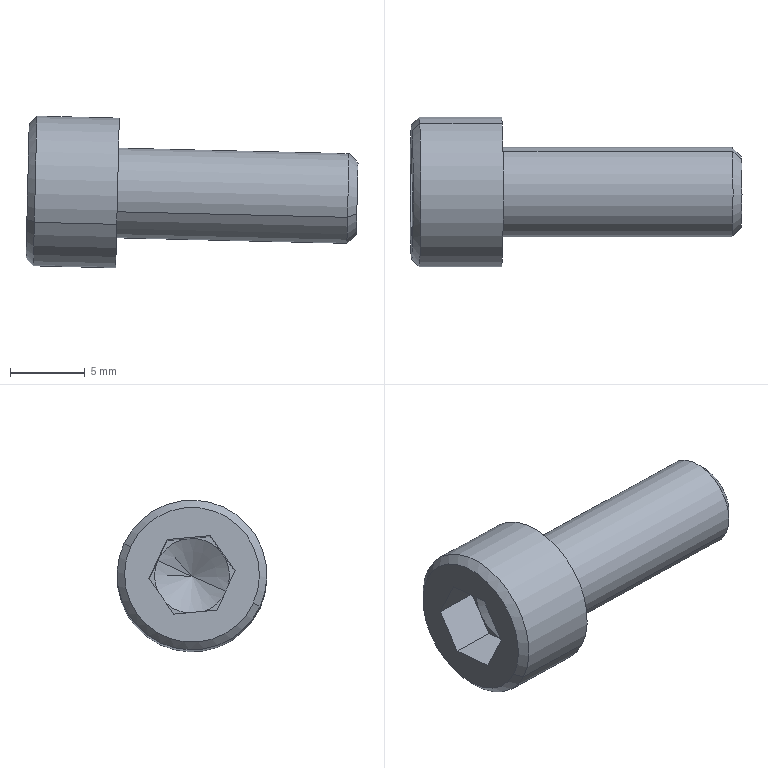Component | SolidWorks | 2012MB0201-1_ASideDoor-1-1_HexSocketHeadCapScrewM6-16FerricOxide-1 | 1 solid | 25 faces | box 22.16 x 10 x 10.13 mm | volume 842 mm3 | plane 15 | cone 6 | cylinder 4 | commonest cylinder face diameters 6 x2 10 x2 | material SCM435
STEP:
#1=CARTESIAN_POINT('',(-48.734,38.787,-7.122));
#2=VERTEX_POINT('',#1);
#3=CARTESIAN_POINT('',(-48.732,38.957,-7.043));
#4=VERTEX_POINT('',#3);
#5=CARTESIAN_POINT('',(-48.733,38.872,-7.083));
#6=DIRECTION('',(0.9997,0.,-0.02392));
#7=DIRECTION('',(0.02173,-0.4184,0.908));
#8=AXIS2_PLACEMENT_3D('',#5,#6,#7);
#9=CIRCLE('',#8,0.0939);
#10=EDGE_CURVE('',#2,#4,#9,.T.);
#11=ORIENTED_EDGE('',*,*,#10,.F.);
#12=CARTESIAN_POINT('',(-48.758,38.765,-7.131));
#13=VERTEX_POINT('',#12);
#14=CARTESIAN_POINT('',(-48.734,38.787,-7.122));
#15=DIRECTION('',(-0.714,-0.6422,-0.2789));
#16=VECTOR('',#15,39.37);
#17=LINE('',#14,#16);
#18=EDGE_CURVE('',#2,#13,#17,.T.);
#19=ORIENTED_EDGE('',*,*,#18,.T.);
#20=CARTESIAN_POINT('',(-48.756,38.979,-7.033));
#21=VERTEX_POINT('',#20);
#22=CARTESIAN_POINT('',(-48.757,38.872,-7.082));
#23=DIRECTION('',(-0.9997,-0.,0.02392));
#24=DIRECTION('',(0.01001,0.9083,0.4183));
#25=AXIS2_PLACEMENT_3D('',#22,#23,#24);
#26=CIRCLE('',#25,0.1181);
#27=EDGE_CURVE('',#21,#13,#26,.T.);
#28=ORIENTED_EDGE('',*,*,#27,.F.);
#29=CARTESIAN_POINT('',(-48.732,38.957,-7.043));
#30=DIRECTION('',(-0.6998,0.6422,0.3127));
#31=VECTOR('',#30,39.37);
#32=LINE('',#29,#31);
#33=EDGE_CURVE('',#4,#21,#32,.T.);
#34=ORIENTED_EDGE('',*,*,#33,.F.);
#35=EDGE_LOOP('',(#11,#19,#28,#34));
#36=FACE_OUTER_BOUND('',#35,.T.);
#37=CARTESIAN_POINT('',(-48.733,38.872,-7.083));
#38=DIRECTION('',(-0.9997,-0.,0.02392));
#39=DIRECTION('',(0.01001,0.9083,0.4183));
#40=AXIS2_PLACEMENT_3D('',#37,#38,#39);
#41=CONICAL_SURFACE('',#40,0.0939,0.7854);
#42=ADVANCED_FACE('',(#36),#41,.T.);
#43=ORIENTED_EDGE('',*,*,#27,.T.);
#44=CARTESIAN_POINT('',(-49.364,38.765,-7.117));
#45=VERTEX_POINT('',#44);
#46=CARTESIAN_POINT('',(-45.428,38.765,-7.211));
#47=DIRECTION('',(-0.9997,-0.,0.02392));
#48=VECTOR('',#47,39.37);
#49=LINE('',#46,#48);
#50=EDGE_CURVE('',#13,#45,#49,.T.);
#51=ORIENTED_EDGE('',*,*,#50,.T.);
#52=CARTESIAN_POINT('',(-49.361,38.979,-7.018));
#53=VERTEX_POINT('',#52);
#54=CARTESIAN_POINT('',(-49.362,38.872,-7.068));
#55=DIRECTION('',(0.9997,0.,-0.02392));
#56=DIRECTION('',(0.01001,0.9083,0.4183));
#57=AXIS2_PLACEMENT_3D('',#54,#55,#56);
#58=CIRCLE('',#57,0.1181);
#59=EDGE_CURVE('',#45,#53,#58,.T.);
#60=ORIENTED_EDGE('',*,*,#59,.T.);
#61=CARTESIAN_POINT('',(-45.425,38.979,-7.112));
#62=DIRECTION('',(-0.9997,-0.,0.02392));
#63=VECTOR('',#62,39.37);
#64=LINE('',#61,#63);
#65=EDGE_CURVE('',#21,#53,#64,.T.);
#66=ORIENTED_EDGE('',*,*,#65,.F.);
#67=EDGE_LOOP('',(#43,#51,#60,#66));
#68=FACE_OUTER_BOUND('',#67,.T.);
#69=CARTESIAN_POINT('',(-45.427,38.872,-7.162));
#70=DIRECTION('',(-0.9997,-0.,0.02392));
#71=DIRECTION('',(0.01001,0.9083,0.4183));
#72=AXIS2_PLACEMENT_3D('',#69,#70,#71);
#73=CYLINDRICAL_SURFACE('',#72,0.1181);
#74=ADVANCED_FACE('',(#68),#73,.T.);
#75=CARTESIAN_POINT('',(-49.36,39.051,-6.985));
#76=VERTEX_POINT('',#75);
#77=CARTESIAN_POINT('',(-49.364,38.693,-7.15));
#78=VERTEX_POINT('',#77);
#79=CARTESIAN_POINT('',(-49.362,38.872,-7.068));
#80=DIRECTION('',(-0.9997,-0.,0.02392));
#81=DIRECTION('',(0.01001,0.9083,0.4183));
#82=AXIS2_PLACEMENT_3D('',#79,#80,#81);
#83=CIRCLE('',#82,0.1969);
#84=EDGE_CURVE('',#76,#78,#83,.T.);
#85=ORIENTED_EDGE('',*,*,#84,.T.);
#86=CARTESIAN_POINT('',(-49.581,38.693,-7.145));
#87=VERTEX_POINT('',#86);
#88=CARTESIAN_POINT('',(-49.364,38.693,-7.15));
#89=DIRECTION('',(-0.9997,-0.,0.02392));
#90=VECTOR('',#89,39.37);
#91=LINE('',#88,#90);
#92=EDGE_CURVE('',#78,#87,#91,.T.);
#93=ORIENTED_EDGE('',*,*,#92,.T.);
#94=CARTESIAN_POINT('',(-49.577,39.051,-6.98));
#95=VERTEX_POINT('',#94);
#96=CARTESIAN_POINT('',(-49.579,38.872,-7.062));
#97=DIRECTION('',(0.9997,0.,-0.02392));
#98=DIRECTION('',(0.01001,0.9083,0.4183));
#99=AXIS2_PLACEMENT_3D('',#96,#97,#98);
#100=CIRCLE('',#99,0.1969);
#101=EDGE_CURVE('',#87,#95,#100,.T.);
#102=ORIENTED_EDGE('',*,*,#101,.T.);
#103=CARTESIAN_POINT('',(-49.36,39.051,-6.985));
#104=DIRECTION('',(-0.9997,-0.,0.02392));
#105=VECTOR('',#104,39.37);
#106=LINE('',#103,#105);
#107=EDGE_CURVE('',#76,#95,#106,.T.);
#108=ORIENTED_EDGE('',*,*,#107,.F.);
#109=EDGE_LOOP('',(#85,#93,#102,#108));
#110=FACE_OUTER_BOUND('',#109,.T.);
#111=CARTESIAN_POINT('',(-49.362,38.872,-7.068));
#112=DIRECTION('',(-0.9997,-0.,0.02392));
#113=DIRECTION('',(0.01001,0.9083,0.4183));
#114=AXIS2_PLACEMENT_3D('',#111,#112,#113);
#115=CYLINDRICAL_SURFACE('',#114,0.1969);
#116=ADVANCED_FACE('',(#110),#115,.T.);
#117=CARTESIAN_POINT('',(-49.6,38.711,-7.136));
#118=VERTEX_POINT('',#117);
#119=CARTESIAN_POINT('',(-49.597,39.033,-6.988));
#120=VERTEX_POINT('',#119);
#121=CARTESIAN_POINT('',(-49.599,38.872,-7.062));
#122=DIRECTION('',(0.9997,0.,-0.02392));
#123=DIRECTION('',(-0.01001,-0.9083,-0.4183));
#124=AXIS2_PLACEMENT_3D('',#121,#122,#123);
#125=CIRCLE('',#124,0.1772);
#126=EDGE_CURVE('',#118,#120,#125,.T.);
#127=ORIENTED_EDGE('',*,*,#126,.T.);
#128=CARTESIAN_POINT('',(-49.577,39.051,-6.98));
#129=DIRECTION('',(0.714,0.6422,0.2789));
#130=VECTOR('',#129,39.37);
#131=LINE('',#128,#130);
#132=EDGE_CURVE('',#120,#95,#131,.T.);
#133=ORIENTED_EDGE('',*,*,#132,.T.);
#134=ORIENTED_EDGE('',*,*,#101,.F.);
#135=CARTESIAN_POINT('',(-49.581,38.693,-7.145));
#136=DIRECTION('',(0.6998,-0.6422,-0.3127));
#137=VECTOR('',#136,39.37);
#138=LINE('',#135,#137);
#139=EDGE_CURVE('',#118,#87,#138,.T.);
#140=ORIENTED_EDGE('',*,*,#139,.F.);
#141=EDGE_LOOP('',(#127,#133,#134,#140));
#142=FACE_OUTER_BOUND('',#141,.T.);
#143=CARTESIAN_POINT('',(-49.579,38.872,-7.062));
#144=DIRECTION('',(0.9997,0.,-0.02392));
#145=DIRECTION('',(-0.01001,-0.9083,-0.4183));
#146=AXIS2_PLACEMENT_3D('',#143,#144,#145);
#147=CONICAL_SURFACE('',#146,0.1969,0.7854);
#148=ADVANCED_FACE('',(#142),#147,.T.);
#149=CARTESIAN_POINT('',(-49.424,38.872,-7.066));
#150=VERTEX_POINT('',#149);
#151=CARTESIAN_POINT('',(-49.48,38.961,-7.024));
#152=VERTEX_POINT('',#151);
#153=CARTESIAN_POINT('',(-49.48,38.961,-7.024));
#154=DIRECTION('',(-0.4912,0.7866,0.3742));
#155=VECTOR('',#154,39.37);
#156=LINE('',#153,#155);
#157=EDGE_CURVE('',#150,#152,#156,.T.);
#158=ORIENTED_EDGE('',*,*,#157,.F.);
#159=CARTESIAN_POINT('',(-49.482,38.783,-7.106));
#160=VERTEX_POINT('',#159);
#161=CARTESIAN_POINT('',(-49.482,38.783,-7.106));
#162=DIRECTION('',(-0.5085,-0.7866,-0.3503));
#163=VECTOR('',#162,39.37);
#164=LINE('',#161,#163);
#165=EDGE_CURVE('',#150,#160,#164,.T.);
#166=ORIENTED_EDGE('',*,*,#165,.T.);
#167=CARTESIAN_POINT('',(-49.479,38.792,-7.008));
#168=VERTEX_POINT('',#167);
#169=CARTESIAN_POINT('',(-49.481,38.872,-7.065));
#170=DIRECTION('',(0.9997,0.,-0.02392));
#171=DIRECTION('',(0.01001,0.9083,0.4183));
#172=AXIS2_PLACEMENT_3D('',#169,#170,#171);
#173=CIRCLE('',#172,0.09843);
#174=EDGE_CURVE('',#168,#160,#173,.T.);
#175=ORIENTED_EDGE('',*,*,#174,.F.);
#176=CARTESIAN_POINT('',(-49.478,38.881,-6.967));
#177=VERTEX_POINT('',#176);
#178=CARTESIAN_POINT('',(-49.481,38.872,-7.065));
#179=DIRECTION('',(0.9997,0.,-0.02392));
#180=DIRECTION('',(0.01001,0.9083,0.4183));
#181=AXIS2_PLACEMENT_3D('',#178,#179,#180);
#182=CIRCLE('',#181,0.09843);
#183=EDGE_CURVE('',#177,#168,#182,.T.);
#184=ORIENTED_EDGE('',*,*,#183,.F.);
#185=CARTESIAN_POINT('',(-49.481,38.872,-7.065));
#186=DIRECTION('',(0.9997,0.,-0.02392));
#187=DIRECTION('',(0.01001,0.9083,0.4183));
#188=AXIS2_PLACEMENT_3D('',#185,#186,#187);
#189=CIRCLE('',#188,0.09843);
#190=EDGE_CURVE('',#152,#177,#189,.T.);
#191=ORIENTED_EDGE('',*,*,#190,.F.);
#192=EDGE_LOOP('',(#158,#166,#175,#184,#191));
#193=FACE_OUTER_BOUND('',#192,.T.);
#194=CARTESIAN_POINT('',(-49.481,38.872,-7.065));
#195=DIRECTION('',(-0.9997,-0.,0.02392));
#196=DIRECTION('',(0.01001,0.9083,0.4183));
#197=AXIS2_PLACEMENT_3D('',#194,#195,#196);
#198=CONICAL_SURFACE('',#197,0.09843,1.047);
#199=ADVANCED_FACE('',(#193),#198,.F.);
#200=ORIENTED_EDGE('',*,*,#50,.F.);
#201=CARTESIAN_POINT('',(-48.757,38.872,-7.082));
#202=DIRECTION('',(-0.9997,-0.,0.02392));
#203=DIRECTION('',(0.01001,0.9083,0.4183));
#204=AXIS2_PLACEMENT_3D('',#201,#202,#203);
#205=CIRCLE('',#204,0.1181);
#206=EDGE_CURVE('',#13,#21,#205,.T.);
#207=ORIENTED_EDGE('',*,*,#206,.T.);
#208=ORIENTED_EDGE('',*,*,#65,.T.);
#209=CARTESIAN_POINT('',(-49.362,38.872,-7.068));
#210=DIRECTION('',(0.9997,0.,-0.02392));
#211=DIRECTION('',(0.01001,0.9083,0.4183));
#212=AXIS2_PLACEMENT_3D('',#209,#210,#211);
#213=CIRCLE('',#212,0.1181);
#214=EDGE_CURVE('',#53,#45,#213,.T.);
#215=ORIENTED_EDGE('',*,*,#214,.T.);
#216=EDGE_LOOP('',(#200,#207,#208,#215));
#217=FACE_OUTER_BOUND('',#216,.T.);
#218=CARTESIAN_POINT('',(-45.427,38.872,-7.162));
#219=DIRECTION('',(-0.9997,-0.,0.02392));
#220=DIRECTION('',(0.01001,0.9083,0.4183));
#221=AXIS2_PLACEMENT_3D('',#218,#219,#220);
#222=CYLINDRICAL_SURFACE('',#221,0.1181);
#223=ADVANCED_FACE('',(#217),#222,.T.);
#224=ORIENTED_EDGE('',*,*,#84,.F.);
#225=CARTESIAN_POINT('',(-49.362,38.872,-7.068));
#226=DIRECTION('',(-0.9997,-0.,0.02392));
#227=DIRECTION('',(0.01001,0.9083,0.4183));
#228=AXIS2_PLACEMENT_3D('',#225,#226,#227);
#229=CIRCLE('',#228,0.1969);
#230=EDGE_CURVE('',#78,#76,#229,.T.);
#231=ORIENTED_EDGE('',*,*,#230,.F.);
#232=EDGE_LOOP('',(#224,#231));
#233=FACE_OUTER_BOUND('',#232,.T.);
#234=ORIENTED_EDGE('',*,*,#214,.F.);
#235=ORIENTED_EDGE('',*,*,#59,.F.);
#236=EDGE_LOOP('',(#234,#235));
#237=FACE_BOUND('',#236,.T.);
#238=CARTESIAN_POINT('',(-49.367,38.954,-7.246));
#239=DIRECTION('',(-0.9997,-0.,0.02392));
#240=DIRECTION('',(0.01001,0.9083,0.4183));
#241=AXIS2_PLACEMENT_3D('',#238,#239,#240);
#242=PLANE('',#241);
#243=ADVANCED_FACE('',(#233,#237),#242,.F.);
#244=ORIENTED_EDGE('',*,*,#92,.F.);
#245=ORIENTED_EDGE('',*,*,#230,.T.);
#246=ORIENTED_EDGE('',*,*,#107,.T.);
#247=CARTESIAN_POINT('',(-49.579,38.872,-7.062));
#248=DIRECTION('',(0.9997,0.,-0.02392));
#249=DIRECTION('',(0.01001,0.9083,0.4183));
#250=AXIS2_PLACEMENT_3D('',#247,#248,#249);
#251=CIRCLE('',#250,0.1969);
#252=EDGE_CURVE('',#95,#87,#251,.T.);
#253=ORIENTED_EDGE('',*,*,#252,.T.);
#254=EDGE_LOOP('',(#244,#245,#246,#253));
#255=FACE_OUTER_BOUND('',#254,.T.);
#256=CARTESIAN_POINT('',(-49.362,38.872,-7.068));
#257=DIRECTION('',(-0.9997,-0.,0.02392));
#258=DIRECTION('',(0.01001,0.9083,0.4183));
#259=AXIS2_PLACEMENT_3D('',#256,#257,#258);
#260=CYLINDRICAL_SURFACE('',#259,0.1969);
#261=ADVANCED_FACE('',(#255),#260,.T.);
#262=ORIENTED_EDGE('',*,*,#132,.F.);
#263=CARTESIAN_POINT('',(-49.599,38.872,-7.062));
#264=DIRECTION('',(0.9997,0.,-0.02392));
#265=DIRECTION('',(-0.01001,-0.9083,-0.4183));
#266=AXIS2_PLACEMENT_3D('',#263,#264,#265);
#267=CIRCLE('',#266,0.1772);
#268=EDGE_CURVE('',#120,#118,#267,.T.);
#269=ORIENTED_EDGE('',*,*,#268,.T.);
#270=ORIENTED_EDGE('',*,*,#139,.T.);
#271=ORIENTED_EDGE('',*,*,#252,.F.);
#272=EDGE_LOOP('',(#262,#269,#270,#271));
#273=FACE_OUTER_BOUND('',#272,.T.);
#274=CARTESIAN_POINT('',(-49.579,38.872,-7.062));
#275=DIRECTION('',(0.9997,0.,-0.02392));
#276=DIRECTION('',(-0.01001,-0.9083,-0.4183));
#277=AXIS2_PLACEMENT_3D('',#274,#275,#276);
#278=CONICAL_SURFACE('',#277,0.1969,0.7854);
#279=ADVANCED_FACE('',(#273),#278,.T.);
#280=CARTESIAN_POINT('',(-49.598,38.759,-7.051));
#281=VERTEX_POINT('',#280);
#282=CARTESIAN_POINT('',(-49.596,38.825,-6.959));
#283=VERTEX_POINT('',#282);
#284=CARTESIAN_POINT('',(-49.598,38.759,-7.051));
#285=DIRECTION('',(0.01953,0.5774,0.8163));
#286=VECTOR('',#285,39.37);
#287=LINE('',#284,#286);
#288=EDGE_CURVE('',#281,#283,#287,.T.);
#289=ORIENTED_EDGE('',*,*,#288,.F.);
#290=CARTESIAN_POINT('',(-49.601,38.806,-7.155));
#291=VERTEX_POINT('',#290);
#292=CARTESIAN_POINT('',(-49.6,38.783,-7.103));
#293=DIRECTION('',(0.02173,-0.4184,0.908));
#294=VECTOR('',#293,39.37);
#295=LINE('',#292,#294);
#296=EDGE_CURVE('',#291,#281,#295,.T.);
#297=ORIENTED_EDGE('',*,*,#296,.F.);
#298=CARTESIAN_POINT('',(-49.601,38.92,-7.165));
#299=VERTEX_POINT('',#298);
#300=CARTESIAN_POINT('',(-49.601,38.92,-7.165));
#301=DIRECTION('',(0.002195,-0.9958,0.09174));
#302=VECTOR('',#301,39.37);
#303=LINE('',#300,#302);
#304=EDGE_CURVE('',#299,#291,#303,.T.);
#305=ORIENTED_EDGE('',*,*,#304,.F.);
#306=CARTESIAN_POINT('',(-49.599,38.985,-7.072));
#307=VERTEX_POINT('',#306);
#308=CARTESIAN_POINT('',(-49.599,38.985,-7.072));
#309=DIRECTION('',(-0.01953,-0.5774,-0.8163));
#310=VECTOR('',#309,39.37);
#311=LINE('',#308,#310);
#312=EDGE_CURVE('',#307,#299,#311,.T.);
#313=ORIENTED_EDGE('',*,*,#312,.F.);
#314=CARTESIAN_POINT('',(-49.596,38.938,-6.969));
#315=VERTEX_POINT('',#314);
#316=CARTESIAN_POINT('',(-49.598,38.961,-7.021));
#317=DIRECTION('',(-0.02173,0.4184,-0.908));
#318=VECTOR('',#317,39.37);
#319=LINE('',#316,#318);
#320=EDGE_CURVE('',#315,#307,#319,.T.);
#321=ORIENTED_EDGE('',*,*,#320,.F.);
#322=CARTESIAN_POINT('',(-49.596,38.825,-6.959));
#323=DIRECTION('',(-0.002195,0.9958,-0.09174));
#324=VECTOR('',#323,39.37);
#325=LINE('',#322,#324);
#326=EDGE_CURVE('',#283,#315,#325,.T.);
#327=ORIENTED_EDGE('',*,*,#326,.F.);
#328=EDGE_LOOP('',(#289,#297,#305,#313,#321,#327));
#329=FACE_BOUND('',#328,.T.);
#330=ORIENTED_EDGE('',*,*,#126,.F.);
#331=ORIENTED_EDGE('',*,*,#268,.F.);
#332=EDGE_LOOP('',(#330,#331));
#333=FACE_OUTER_BOUND('',#332,.T.);
#334=CARTESIAN_POINT('',(-49.599,38.872,-7.062));
#335=DIRECTION('',(0.9997,0.,-0.02392));
#336=DIRECTION('',(-0.01001,-0.9083,-0.4183));
#337=AXIS2_PLACEMENT_3D('',#334,#335,#336);
#338=PLANE('',#337);
#339=ADVANCED_FACE('',(#329,#333),#338,.F.);
#340=CARTESIAN_POINT('',(-49.478,38.938,-6.972));
#341=VERTEX_POINT('',#340);
#342=CARTESIAN_POINT('',(-49.478,38.938,-6.972));
#343=DIRECTION('',(-0.9997,-0.,0.02392));
#344=VECTOR('',#343,39.37);
#345=LINE('',#342,#344);
#346=EDGE_CURVE('',#341,#315,#345,.T.);
#347=ORIENTED_EDGE('',*,*,#346,.F.);
#348=CARTESIAN_POINT('',(-49.478,38.881,-6.967));
#349=DIRECTION('',(-0.002195,0.9958,-0.09174));
#350=VECTOR('',#349,39.37);
#351=LINE('',#348,#350);
#352=EDGE_CURVE('',#177,#341,#351,.T.);
#353=ORIENTED_EDGE('',*,*,#352,.F.);
#354=CARTESIAN_POINT('',(-49.478,38.825,-6.962));
#355=VERTEX_POINT('',#354);
#356=CARTESIAN_POINT('',(-49.478,38.825,-6.962));
#357=DIRECTION('',(-0.002195,0.9958,-0.09174));
#358=VECTOR('',#357,39.37);
#359=LINE('',#356,#358);
#360=EDGE_CURVE('',#355,#177,#359,.T.);
#361=ORIENTED_EDGE('',*,*,#360,.F.);
#362=CARTESIAN_POINT('',(-49.478,38.825,-6.962));
#363=DIRECTION('',(0.9997,0.,-0.02392));
#364=VECTOR('',#363,39.37);
#365=LINE('',#362,#364);
#366=EDGE_CURVE('',#283,#355,#365,.T.);
#367=ORIENTED_EDGE('',*,*,#366,.F.);
#368=ORIENTED_EDGE('',*,*,#326,.T.);
#369=EDGE_LOOP('',(#347,#353,#361,#367,#368));
#370=FACE_OUTER_BOUND('',#369,.T.);
#371=CARTESIAN_POINT('',(-49.478,38.825,-6.962));
#372=DIRECTION('',(0.02382,0.09177,0.9955));
#373=DIRECTION('',(-0.002195,0.9958,-0.09174));
#374=AXIS2_PLACEMENT_3D('',#371,#372,#373);
#375=PLANE('',#374);
#376=ADVANCED_FACE('',(#370),#375,.F.);
#377=ORIENTED_EDGE('',*,*,#366,.T.);
#378=CARTESIAN_POINT('',(-49.479,38.792,-7.008));
#379=DIRECTION('',(0.01953,0.5774,0.8163));
#380=VECTOR('',#379,39.37);
#381=LINE('',#378,#380);
#382=EDGE_CURVE('',#168,#355,#381,.T.);
#383=ORIENTED_EDGE('',*,*,#382,.F.);
#384=CARTESIAN_POINT('',(-49.48,38.759,-7.054));
#385=VERTEX_POINT('',#384);
#386=CARTESIAN_POINT('',(-49.48,38.759,-7.054));
#387=DIRECTION('',(0.01953,0.5774,0.8163));
#388=VECTOR('',#387,39.37);
#389=LINE('',#386,#388);
#390=EDGE_CURVE('',#385,#168,#389,.T.);
#391=ORIENTED_EDGE('',*,*,#390,.F.);
#392=CARTESIAN_POINT('',(-49.48,38.759,-7.054));
#393=DIRECTION('',(0.9997,0.,-0.02392));
#394=VECTOR('',#393,39.37);
#395=LINE('',#392,#394);
#396=EDGE_CURVE('',#281,#385,#395,.T.);
#397=ORIENTED_EDGE('',*,*,#396,.F.);
#398=ORIENTED_EDGE('',*,*,#288,.T.);
#399=EDGE_LOOP('',(#377,#383,#391,#397,#398));
#400=FACE_OUTER_BOUND('',#399,.T.);
#401=CARTESIAN_POINT('',(-49.48,38.759,-7.054));
#402=DIRECTION('',(0.01381,-0.8165,0.5772));
#403=DIRECTION('',(0.01953,0.5774,0.8163));
#404=AXIS2_PLACEMENT_3D('',#401,#402,#403);
#405=PLANE('',#404);
#406=ADVANCED_FACE('',(#400),#405,.F.);
#407=ORIENTED_EDGE('',*,*,#396,.T.);
#408=CARTESIAN_POINT('',(-49.482,38.783,-7.106));
#409=DIRECTION('',(0.02173,-0.4184,0.908));
#410=VECTOR('',#409,39.37);
#411=LINE('',#408,#410);
#412=EDGE_CURVE('',#160,#385,#411,.T.);
#413=ORIENTED_EDGE('',*,*,#412,.F.);
#414=CARTESIAN_POINT('',(-49.483,38.806,-7.158));
#415=VERTEX_POINT('',#414);
#416=CARTESIAN_POINT('',(-49.482,38.783,-7.106));
#417=DIRECTION('',(0.02173,-0.4184,0.908));
#418=VECTOR('',#417,39.37);
#419=LINE('',#416,#418);
#420=EDGE_CURVE('',#415,#160,#419,.T.);
#421=ORIENTED_EDGE('',*,*,#420,.F.);
#422=CARTESIAN_POINT('',(-49.483,38.806,-7.158));
#423=DIRECTION('',(0.9997,0.,-0.02392));
#424=VECTOR('',#423,39.37);
#425=LINE('',#422,#424);
#426=EDGE_CURVE('',#291,#415,#425,.T.);
#427=ORIENTED_EDGE('',*,*,#426,.F.);
#428=ORIENTED_EDGE('',*,*,#296,.T.);
#429=EDGE_LOOP('',(#407,#413,#421,#427,#428));
#430=FACE_OUTER_BOUND('',#429,.T.);
#431=CARTESIAN_POINT('',(-49.483,38.806,-7.158));
#432=DIRECTION('',(-0.01001,-0.9083,-0.4183));
#433=DIRECTION('',(-0.9997,-0.,0.02392));
#434=AXIS2_PLACEMENT_3D('',#431,#432,#433);
#435=PLANE('',#434);
#436=ADVANCED_FACE('',(#430),#435,.F.);
#437=ORIENTED_EDGE('',*,*,#426,.T.);
#438=CARTESIAN_POINT('',(-49.483,38.863,-7.163));
#439=VERTEX_POINT('',#438);
#440=CARTESIAN_POINT('',(-49.483,38.863,-7.163));
#441=DIRECTION('',(0.002195,-0.9958,0.09174));
#442=VECTOR('',#441,39.37);
#443=LINE('',#440,#442);
#444=EDGE_CURVE('',#439,#415,#443,.T.);
#445=ORIENTED_EDGE('',*,*,#444,.F.);
#446=CARTESIAN_POINT('',(-49.483,38.92,-7.168));
#447=VERTEX_POINT('',#446);
#448=CARTESIAN_POINT('',(-49.483,38.92,-7.168));
#449=DIRECTION('',(0.002195,-0.9958,0.09174));
#450=VECTOR('',#449,39.37);
#451=LINE('',#448,#450);
#452=EDGE_CURVE('',#447,#439,#451,.T.);
#453=ORIENTED_EDGE('',*,*,#452,.F.);
#454=CARTESIAN_POINT('',(-49.483,38.92,-7.168));
#455=DIRECTION('',(0.9997,0.,-0.02392));
#456=VECTOR('',#455,39.37);
#457=LINE('',#454,#456);
#458=EDGE_CURVE('',#299,#447,#457,.T.);
#459=ORIENTED_EDGE('',*,*,#458,.F.);
#460=ORIENTED_EDGE('',*,*,#304,.T.);
#461=EDGE_LOOP('',(#437,#445,#453,#459,#460));
#462=FACE_OUTER_BOUND('',#461,.T.);
#463=CARTESIAN_POINT('',(-49.483,38.92,-7.168));
#464=DIRECTION('',(-0.02382,-0.09177,-0.9955));
#465=DIRECTION('',(0.002195,-0.9958,0.09174));
#466=AXIS2_PLACEMENT_3D('',#463,#464,#465);
#467=PLANE('',#466);
#468=ADVANCED_FACE('',(#462),#467,.F.);
#469=ORIENTED_EDGE('',*,*,#458,.T.);
#470=CARTESIAN_POINT('',(-49.482,38.952,-7.122));
#471=VERTEX_POINT('',#470);
#472=CARTESIAN_POINT('',(-49.482,38.952,-7.122));
#473=DIRECTION('',(-0.01953,-0.5774,-0.8163));
#474=VECTOR('',#473,39.37);
#475=LINE('',#472,#474);
#476=EDGE_CURVE('',#471,#447,#475,.T.);
#477=ORIENTED_EDGE('',*,*,#476,.F.);
#478=CARTESIAN_POINT('',(-49.481,38.985,-7.075));
#479=VERTEX_POINT('',#478);
#480=CARTESIAN_POINT('',(-49.481,38.985,-7.075));
#481=DIRECTION('',(-0.01953,-0.5774,-0.8163));
#482=VECTOR('',#481,39.37);
#483=LINE('',#480,#482);
#484=EDGE_CURVE('',#479,#471,#483,.T.);
#485=ORIENTED_EDGE('',*,*,#484,.F.);
#486=CARTESIAN_POINT('',(-49.481,38.985,-7.075));
#487=DIRECTION('',(0.9997,0.,-0.02392));
#488=VECTOR('',#487,39.37);
#489=LINE('',#486,#488);
#490=EDGE_CURVE('',#307,#479,#489,.T.);
#491=ORIENTED_EDGE('',*,*,#490,.F.);
#492=ORIENTED_EDGE('',*,*,#312,.T.);
#493=EDGE_LOOP('',(#469,#477,#485,#491,#492));
#494=FACE_OUTER_BOUND('',#493,.T.);
#495=CARTESIAN_POINT('',(-49.481,38.985,-7.075));
#496=DIRECTION('',(-0.01381,0.8165,-0.5772));
#497=DIRECTION('',(-0.01953,-0.5774,-0.8163));
#498=AXIS2_PLACEMENT_3D('',#495,#496,#497);
#499=PLANE('',#498);
#500=ADVANCED_FACE('',(#494),#499,.F.);
#501=ORIENTED_EDGE('',*,*,#490,.T.);
#502=CARTESIAN_POINT('',(-49.478,38.938,-6.972));
#503=DIRECTION('',(-0.02173,0.4184,-0.908));
#504=VECTOR('',#503,39.37);
#505=LINE('',#502,#504);
#506=EDGE_CURVE('',#152,#479,#505,.T.);
#507=ORIENTED_EDGE('',*,*,#506,.F.);
#508=CARTESIAN_POINT('',(-49.48,38.961,-7.024));
#509=DIRECTION('',(-0.02173,0.4184,-0.908));
#510=VECTOR('',#509,39.37);
#511=LINE('',#508,#510);
#512=EDGE_CURVE('',#341,#152,#511,.T.);
#513=ORIENTED_EDGE('',*,*,#512,.F.);
#514=ORIENTED_EDGE('',*,*,#346,.T.);
#515=ORIENTED_EDGE('',*,*,#320,.T.);
#516=EDGE_LOOP('',(#501,#507,#513,#514,#515));
#517=FACE_OUTER_BOUND('',#516,.T.);
#518=CARTESIAN_POINT('',(-49.478,38.938,-6.972));
#519=DIRECTION('',(0.01001,0.9083,0.4183));
#520=DIRECTION('',(0.9997,0.,-0.02392));
#521=AXIS2_PLACEMENT_3D('',#518,#519,#520);
#522=PLANE('',#521);
#523=ADVANCED_FACE('',(#517),#522,.F.);
#524=CARTESIAN_POINT('',(-49.481,38.872,-7.065));
#525=DIRECTION('',(0.9997,0.,-0.02392));
#526=DIRECTION('',(0.01001,0.9083,0.4183));
#527=AXIS2_PLACEMENT_3D('',#524,#525,#526);
#528=CIRCLE('',#527,0.09843);
#529=EDGE_CURVE('',#471,#152,#528,.T.);
#530=ORIENTED_EDGE('',*,*,#529,.T.);
#531=ORIENTED_EDGE('',*,*,#506,.T.);
#532=ORIENTED_EDGE('',*,*,#484,.T.);
#533=EDGE_LOOP('',(#530,#531,#532));
#534=FACE_OUTER_BOUND('',#533,.T.);
#535=CARTESIAN_POINT('',(-49.481,38.872,-7.065));
#536=DIRECTION('',(-0.9997,-0.,0.02392));
#537=DIRECTION('',(0.01001,0.9083,0.4183));
#538=AXIS2_PLACEMENT_3D('',#535,#536,#537);
#539=PLANE('',#538);
#540=ADVANCED_FACE('',(#534),#539,.T.);
#541=ORIENTED_EDGE('',*,*,#165,.F.);
#542=ORIENTED_EDGE('',*,*,#157,.T.);
#543=ORIENTED_EDGE('',*,*,#529,.F.);
#544=CARTESIAN_POINT('',(-49.481,38.872,-7.065));
#545=DIRECTION('',(0.9997,0.,-0.02392));
#546=DIRECTION('',(0.01001,0.9083,0.4183));
#547=AXIS2_PLACEMENT_3D('',#544,#545,#546);
#548=CIRCLE('',#547,0.09843);
#549=EDGE_CURVE('',#439,#471,#548,.T.);
#550=ORIENTED_EDGE('',*,*,#549,.F.);
#551=CARTESIAN_POINT('',(-49.481,38.872,-7.065));
#552=DIRECTION('',(0.9997,0.,-0.02392));
#553=DIRECTION('',(0.01001,0.9083,0.4183));
#554=AXIS2_PLACEMENT_3D('',#551,#552,#553);
#555=CIRCLE('',#554,0.09843);
#556=EDGE_CURVE('',#160,#439,#555,.T.);
#557=ORIENTED_EDGE('',*,*,#556,.F.);
#558=EDGE_LOOP('',(#541,#542,#543,#550,#557));
#559=FACE_OUTER_BOUND('',#558,.T.);
#560=CARTESIAN_POINT('',(-49.481,38.872,-7.065));
#561=DIRECTION('',(-0.9997,-0.,0.02392));
#562=DIRECTION('',(0.01001,0.9083,0.4183));
#563=AXIS2_PLACEMENT_3D('',#560,#561,#562);
#564=CONICAL_SURFACE('',#563,0.09843,1.047);
#565=ADVANCED_FACE('',(#559),#564,.F.);
#566=ORIENTED_EDGE('',*,*,#549,.T.);
#567=ORIENTED_EDGE('',*,*,#476,.T.);
#568=ORIENTED_EDGE('',*,*,#452,.T.);
#569=EDGE_LOOP('',(#566,#567,#568));
#570=FACE_OUTER_BOUND('',#569,.T.);
#571=CARTESIAN_POINT('',(-49.481,38.872,-7.065));
#572=DIRECTION('',(-0.9997,-0.,0.02392));
#573=DIRECTION('',(0.01001,0.9083,0.4183));
#574=AXIS2_PLACEMENT_3D('',#571,#572,#573);
#575=PLANE('',#574);
#576=ADVANCED_FACE('',(#570),#575,.T.);
#577=ORIENTED_EDGE('',*,*,#556,.T.);
#578=ORIENTED_EDGE('',*,*,#444,.T.);
#579=ORIENTED_EDGE('',*,*,#420,.T.);
#580=EDGE_LOOP('',(#577,#578,#579));
#581=FACE_OUTER_BOUND('',#580,.T.);
#582=CARTESIAN_POINT('',(-49.481,38.872,-7.065));
#583=DIRECTION('',(-0.9997,-0.,0.02392));
#584=DIRECTION('',(0.01001,0.9083,0.4183));
#585=AXIS2_PLACEMENT_3D('',#582,#583,#584);
#586=PLANE('',#585);
#587=ADVANCED_FACE('',(#581),#586,.T.);
#588=ORIENTED_EDGE('',*,*,#174,.T.);
#589=ORIENTED_EDGE('',*,*,#412,.T.);
#590=ORIENTED_EDGE('',*,*,#390,.T.);
#591=EDGE_LOOP('',(#588,#589,#590));
#592=FACE_OUTER_BOUND('',#591,.T.);
#593=CARTESIAN_POINT('',(-49.481,38.872,-7.065));
#594=DIRECTION('',(-0.9997,-0.,0.02392));
#595=DIRECTION('',(0.01001,0.9083,0.4183));
#596=AXIS2_PLACEMENT_3D('',#593,#594,#595);
#597=PLANE('',#596);
#598=ADVANCED_FACE('',(#592),#597,.T.);
#599=ORIENTED_EDGE('',*,*,#183,.T.);
#600=ORIENTED_EDGE('',*,*,#382,.T.);
#601=ORIENTED_EDGE('',*,*,#360,.T.);
#602=EDGE_LOOP('',(#599,#600,#601));
#603=FACE_OUTER_BOUND('',#602,.T.);
#604=CARTESIAN_POINT('',(-49.481,38.872,-7.065));
#605=DIRECTION('',(-0.9997,-0.,0.02392));
#606=DIRECTION('',(0.01001,0.9083,0.4183));
#607=AXIS2_PLACEMENT_3D('',#604,#605,#606);
#608=PLANE('',#607);
#609=ADVANCED_FACE('',(#603),#608,.T.);
#610=ORIENTED_EDGE('',*,*,#190,.T.);
#611=ORIENTED_EDGE('',*,*,#352,.T.);
#612=ORIENTED_EDGE('',*,*,#512,.T.);
#613=EDGE_LOOP('',(#610,#611,#612));
#614=FACE_OUTER_BOUND('',#613,.T.);
#615=CARTESIAN_POINT('',(-49.481,38.872,-7.065));
#616=DIRECTION('',(-0.9997,-0.,0.02392));
#617=DIRECTION('',(0.01001,0.9083,0.4183));
#618=AXIS2_PLACEMENT_3D('',#615,#616,#617);
#619=PLANE('',#618);
#620=ADVANCED_FACE('',(#614),#619,.T.);
#621=CARTESIAN_POINT('',(-48.733,38.872,-7.083));
#622=DIRECTION('',(0.9997,0.,-0.02392));
#623=DIRECTION('',(0.02173,-0.4184,0.908));
#624=AXIS2_PLACEMENT_3D('',#621,#622,#623);
#625=CIRCLE('',#624,0.0939);
#626=EDGE_CURVE('',#4,#2,#625,.T.);
#627=ORIENTED_EDGE('',*,*,#626,.T.);
#628=ORIENTED_EDGE('',*,*,#10,.T.);
#629=EDGE_LOOP('',(#627,#628));
#630=FACE_OUTER_BOUND('',#629,.T.);
#631=CARTESIAN_POINT('',(-48.744,38.868,-7.545));
#632=DIRECTION('',(-0.9997,-0.,0.02392));
#633=DIRECTION('',(0.02173,-0.4184,0.908));
#634=AXIS2_PLACEMENT_3D('',#631,#632,#633);
#635=PLANE('',#634);
#636=ADVANCED_FACE('',(#630),#635,.F.);
#637=ORIENTED_EDGE('',*,*,#18,.F.);
#638=ORIENTED_EDGE('',*,*,#626,.F.);
#639=ORIENTED_EDGE('',*,*,#33,.T.);
#640=ORIENTED_EDGE('',*,*,#206,.F.);
#641=EDGE_LOOP('',(#637,#638,#639,#640));
#642=FACE_OUTER_BOUND('',#641,.T.);
#643=CARTESIAN_POINT('',(-48.733,38.872,-7.083));
#644=DIRECTION('',(-0.9997,-0.,0.02392));
#645=DIRECTION('',(0.01001,0.9083,0.4183));
#646=AXIS2_PLACEMENT_3D('',#643,#644,#645);
#647=CONICAL_SURFACE('',#646,0.0939,0.7854);
#648=ADVANCED_FACE('',(#642),#647,.T.);
#649=CLOSED_SHELL('',(#42,#74,#116,#148,#199,#223,#243,#261,#279,#339,#376,#406,#436,#468,#500,#523,#540,#565,#576,#587,#598,#609,#620,#636,#648));
#650=MANIFOLD_SOLID_BREP('',#649);
#651=CARTESIAN_POINT('',(0.,0.,0.));
#652=DIRECTION('',(0.,0.,1.));
#653=DIRECTION('',(1.,0.,0.));
#654=AXIS2_PLACEMENT_3D('',#651,#652,#653);
#655=(LENGTH_UNIT()NAMED_UNIT(*)SI_UNIT($,.METRE.));
#656=LENGTH_MEASURE_WITH_UNIT(LENGTH_MEASURE(0.0254),#655);
#657=DIMENSIONAL_EXPONENTS(1.,0.,0.,0.,0.,0.,0.);
#658=(CONVERSION_BASED_UNIT('',#656)LENGTH_UNIT()NAMED_UNIT(#657));
#659=UNCERTAINTY_MEASURE_WITH_UNIT(LENGTH_MEASURE(0.00001),#658,'','');
#660=(NAMED_UNIT(*)PLANE_ANGLE_UNIT()SI_UNIT($,.RADIAN.));
#661=(NAMED_UNIT(*)SI_UNIT($,.STERADIAN.)SOLID_ANGLE_UNIT());
#662=(GEOMETRIC_REPRESENTATION_CONTEXT(3)GLOBAL_UNCERTAINTY_ASSIGNED_CONTEXT((#659))GLOBAL_UNIT_ASSIGNED_CONTEXT((#658,#660,#661))REPRESENTATION_CONTEXT('',''));
#663=ADVANCED_BREP_SHAPE_REPRESENTATION('',(#650,#654),#662);
#664=COLOUR_RGB('',0.7922,0.8196,0.9333);
#665=FILL_AREA_STYLE_COLOUR('',#664);
#666=FILL_AREA_STYLE('',(#665));
#667=SURFACE_STYLE_FILL_AREA(#666);
#668=SURFACE_SIDE_STYLE('',(#667));
#669=SURFACE_STYLE_USAGE(.BOTH.,#668);
#670=PRESENTATION_STYLE_ASSIGNMENT((#669));
#671=STYLED_ITEM('',(#670),#650);
#672=(LENGTH_UNIT()NAMED_UNIT(*)SI_UNIT($,.METRE.));
#673=LENGTH_MEASURE_WITH_UNIT(LENGTH_MEASURE(0.0254),#672);
#674=DIMENSIONAL_EXPONENTS(1.,0.,0.,0.,0.,0.,0.);
#675=(CONVERSION_BASED_UNIT('',#673)LENGTH_UNIT()NAMED_UNIT(#674));
#676=UNCERTAINTY_MEASURE_WITH_UNIT(LENGTH_MEASURE(0.00001),#675,'','');
#677=(NAMED_UNIT(*)PLANE_ANGLE_UNIT()SI_UNIT($,.RADIAN.));
#678=(NAMED_UNIT(*)SI_UNIT($,.STERADIAN.)SOLID_ANGLE_UNIT());
#679=(GEOMETRIC_REPRESENTATION_CONTEXT(3)GLOBAL_UNCERTAINTY_ASSIGNED_CONTEXT((#676))GLOBAL_UNIT_ASSIGNED_CONTEXT((#675,#677,#678))REPRESENTATION_CONTEXT('',''));
#680=MECHANICAL_DESIGN_GEOMETRIC_PRESENTATION_REPRESENTATION('',(#671),#679);
#681=PRESENTATION_LAYER_ASSIGNMENT('','',(#671));